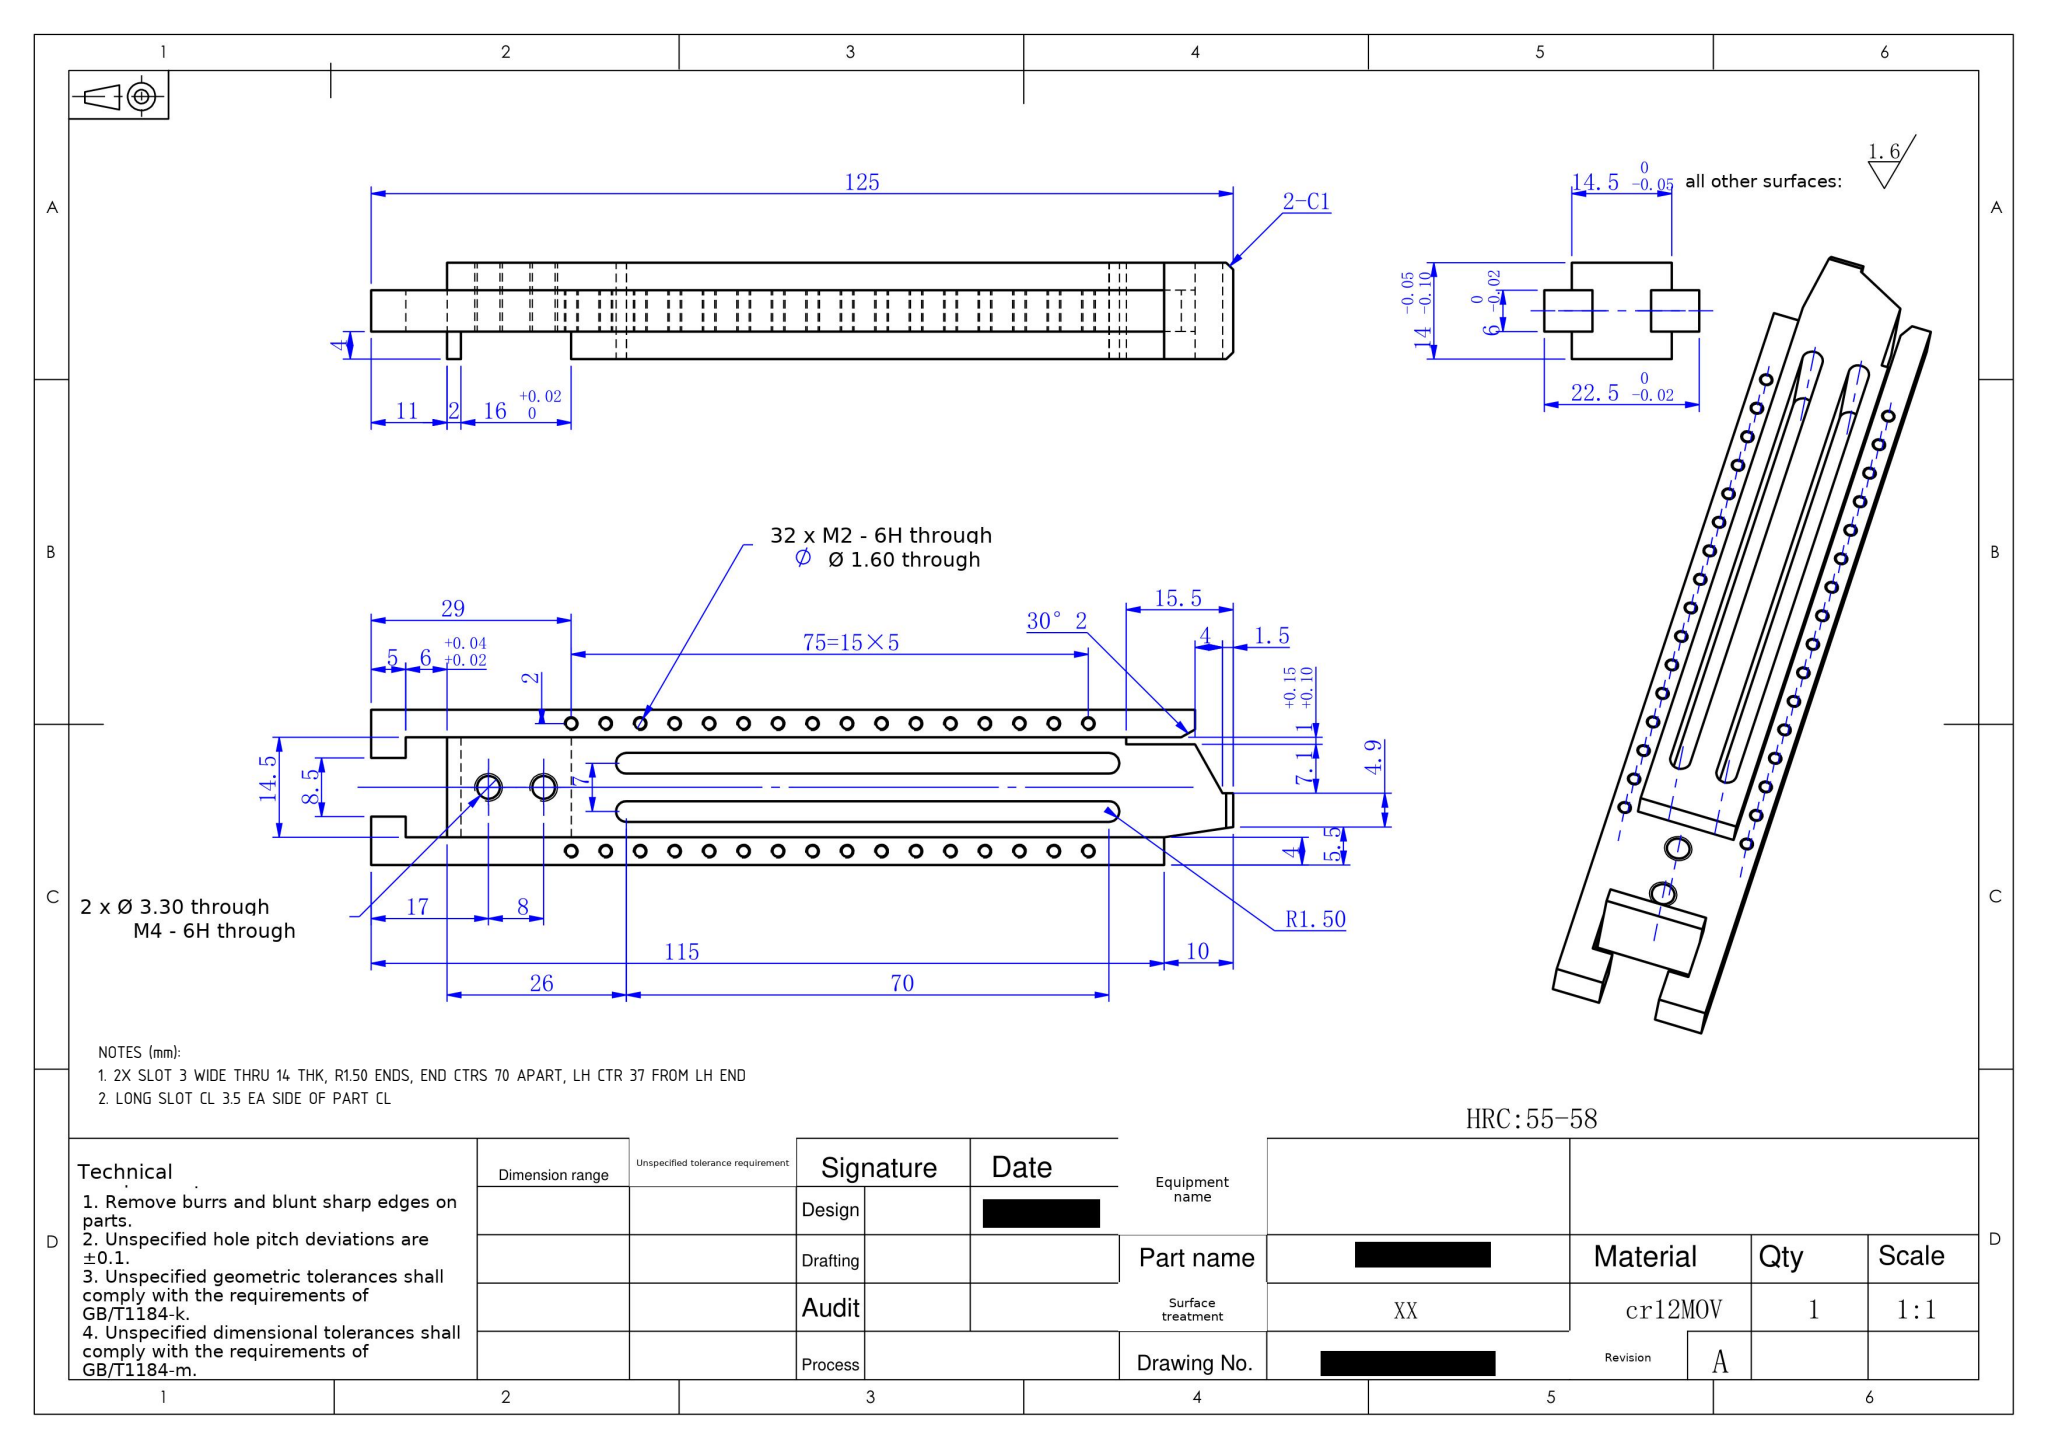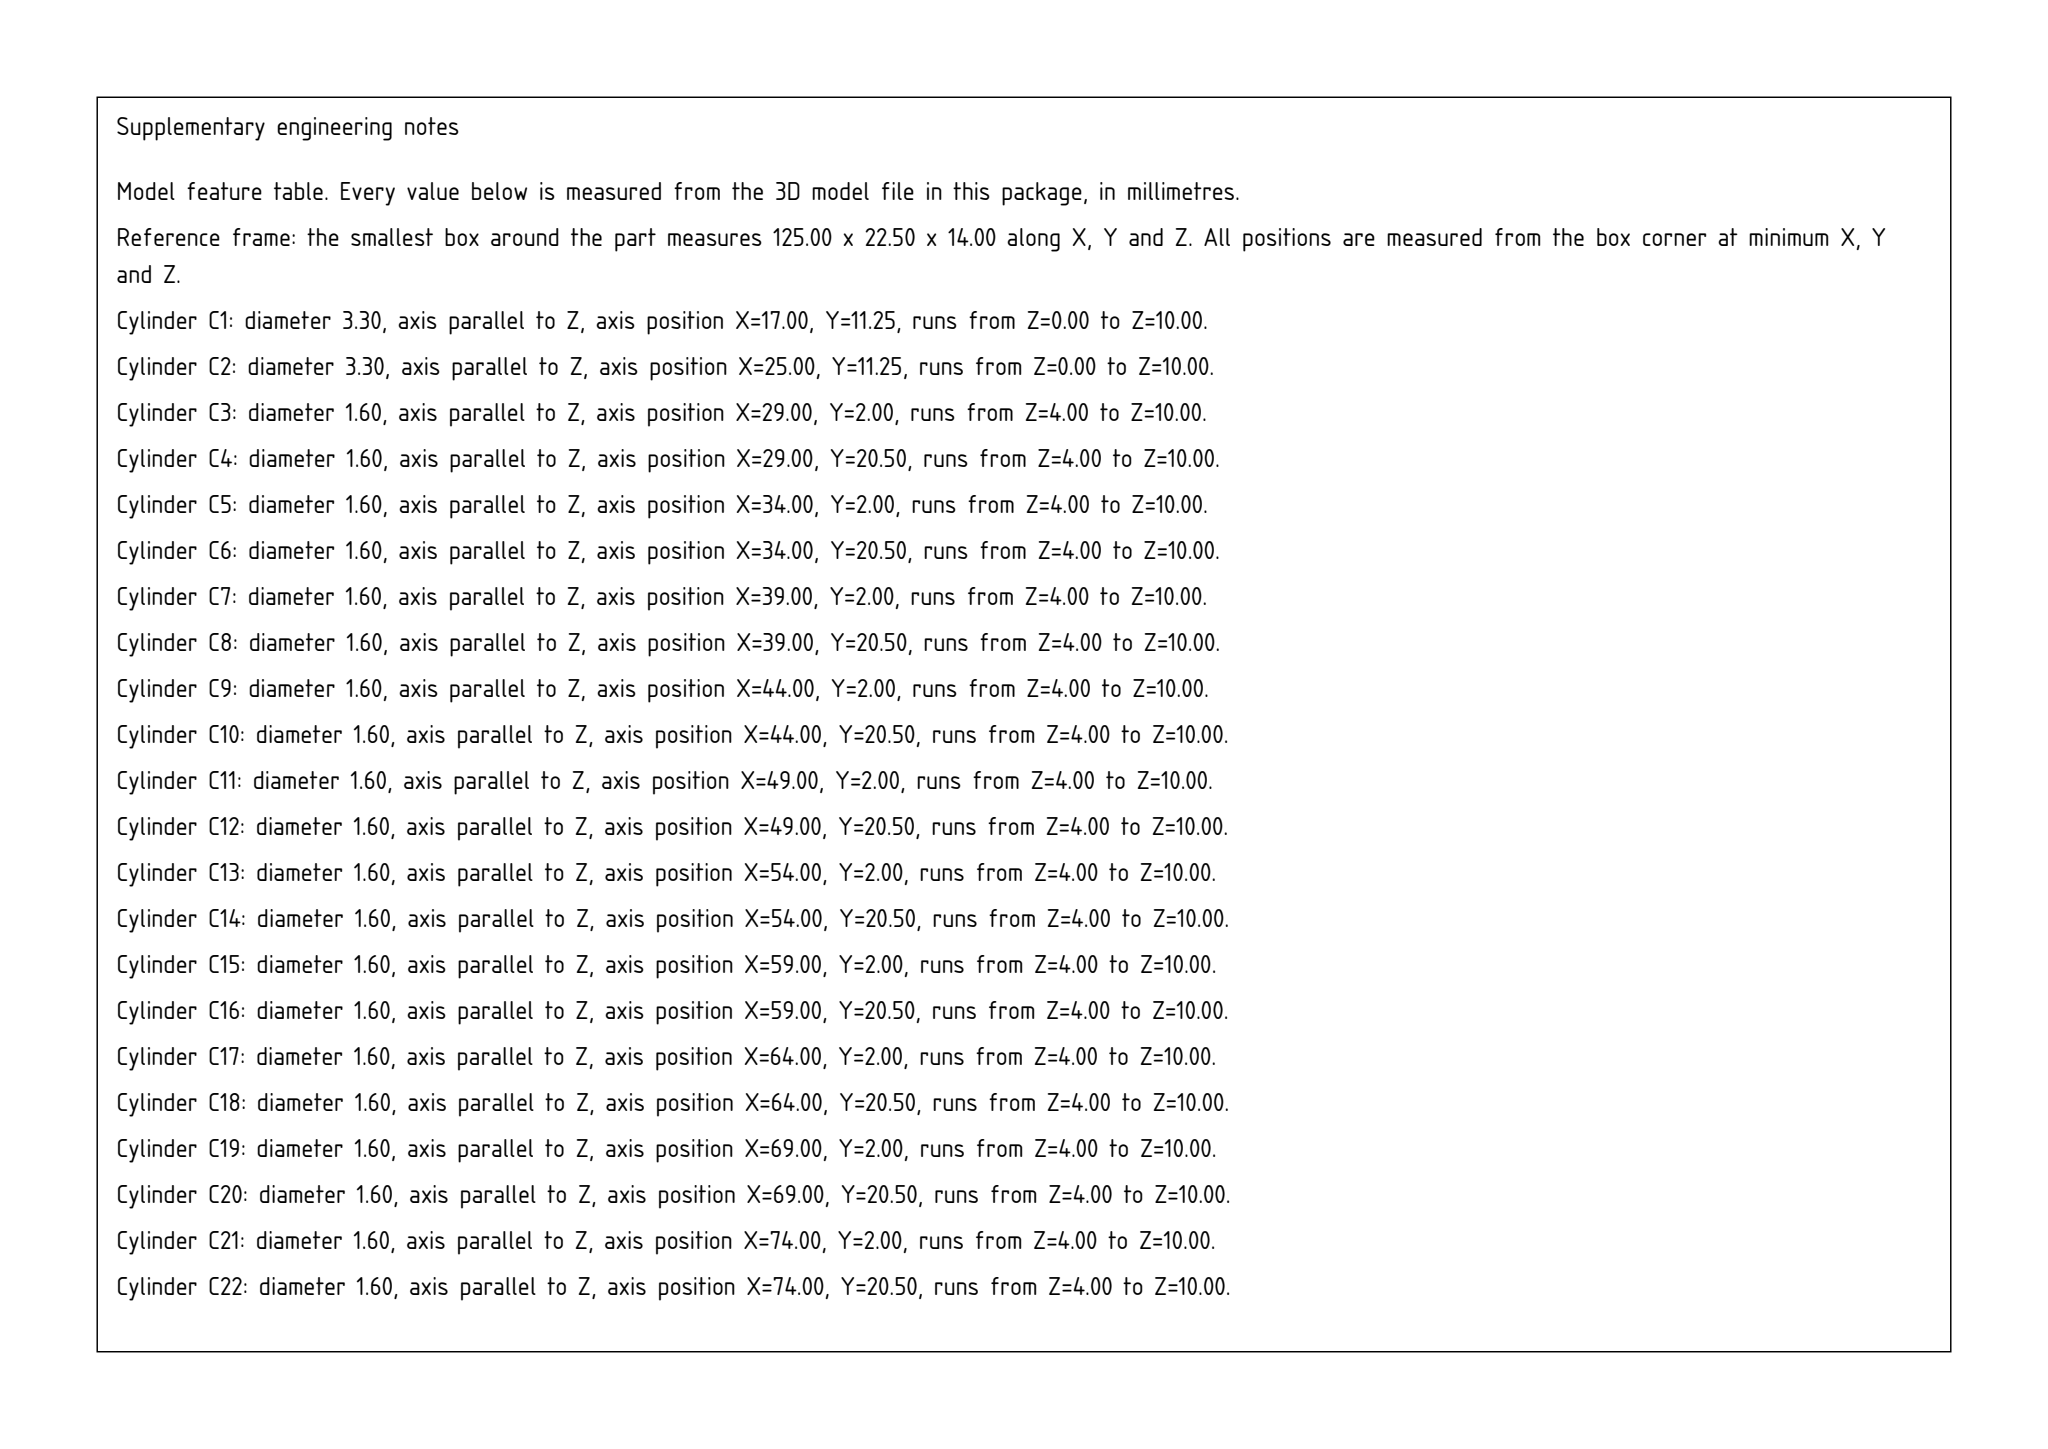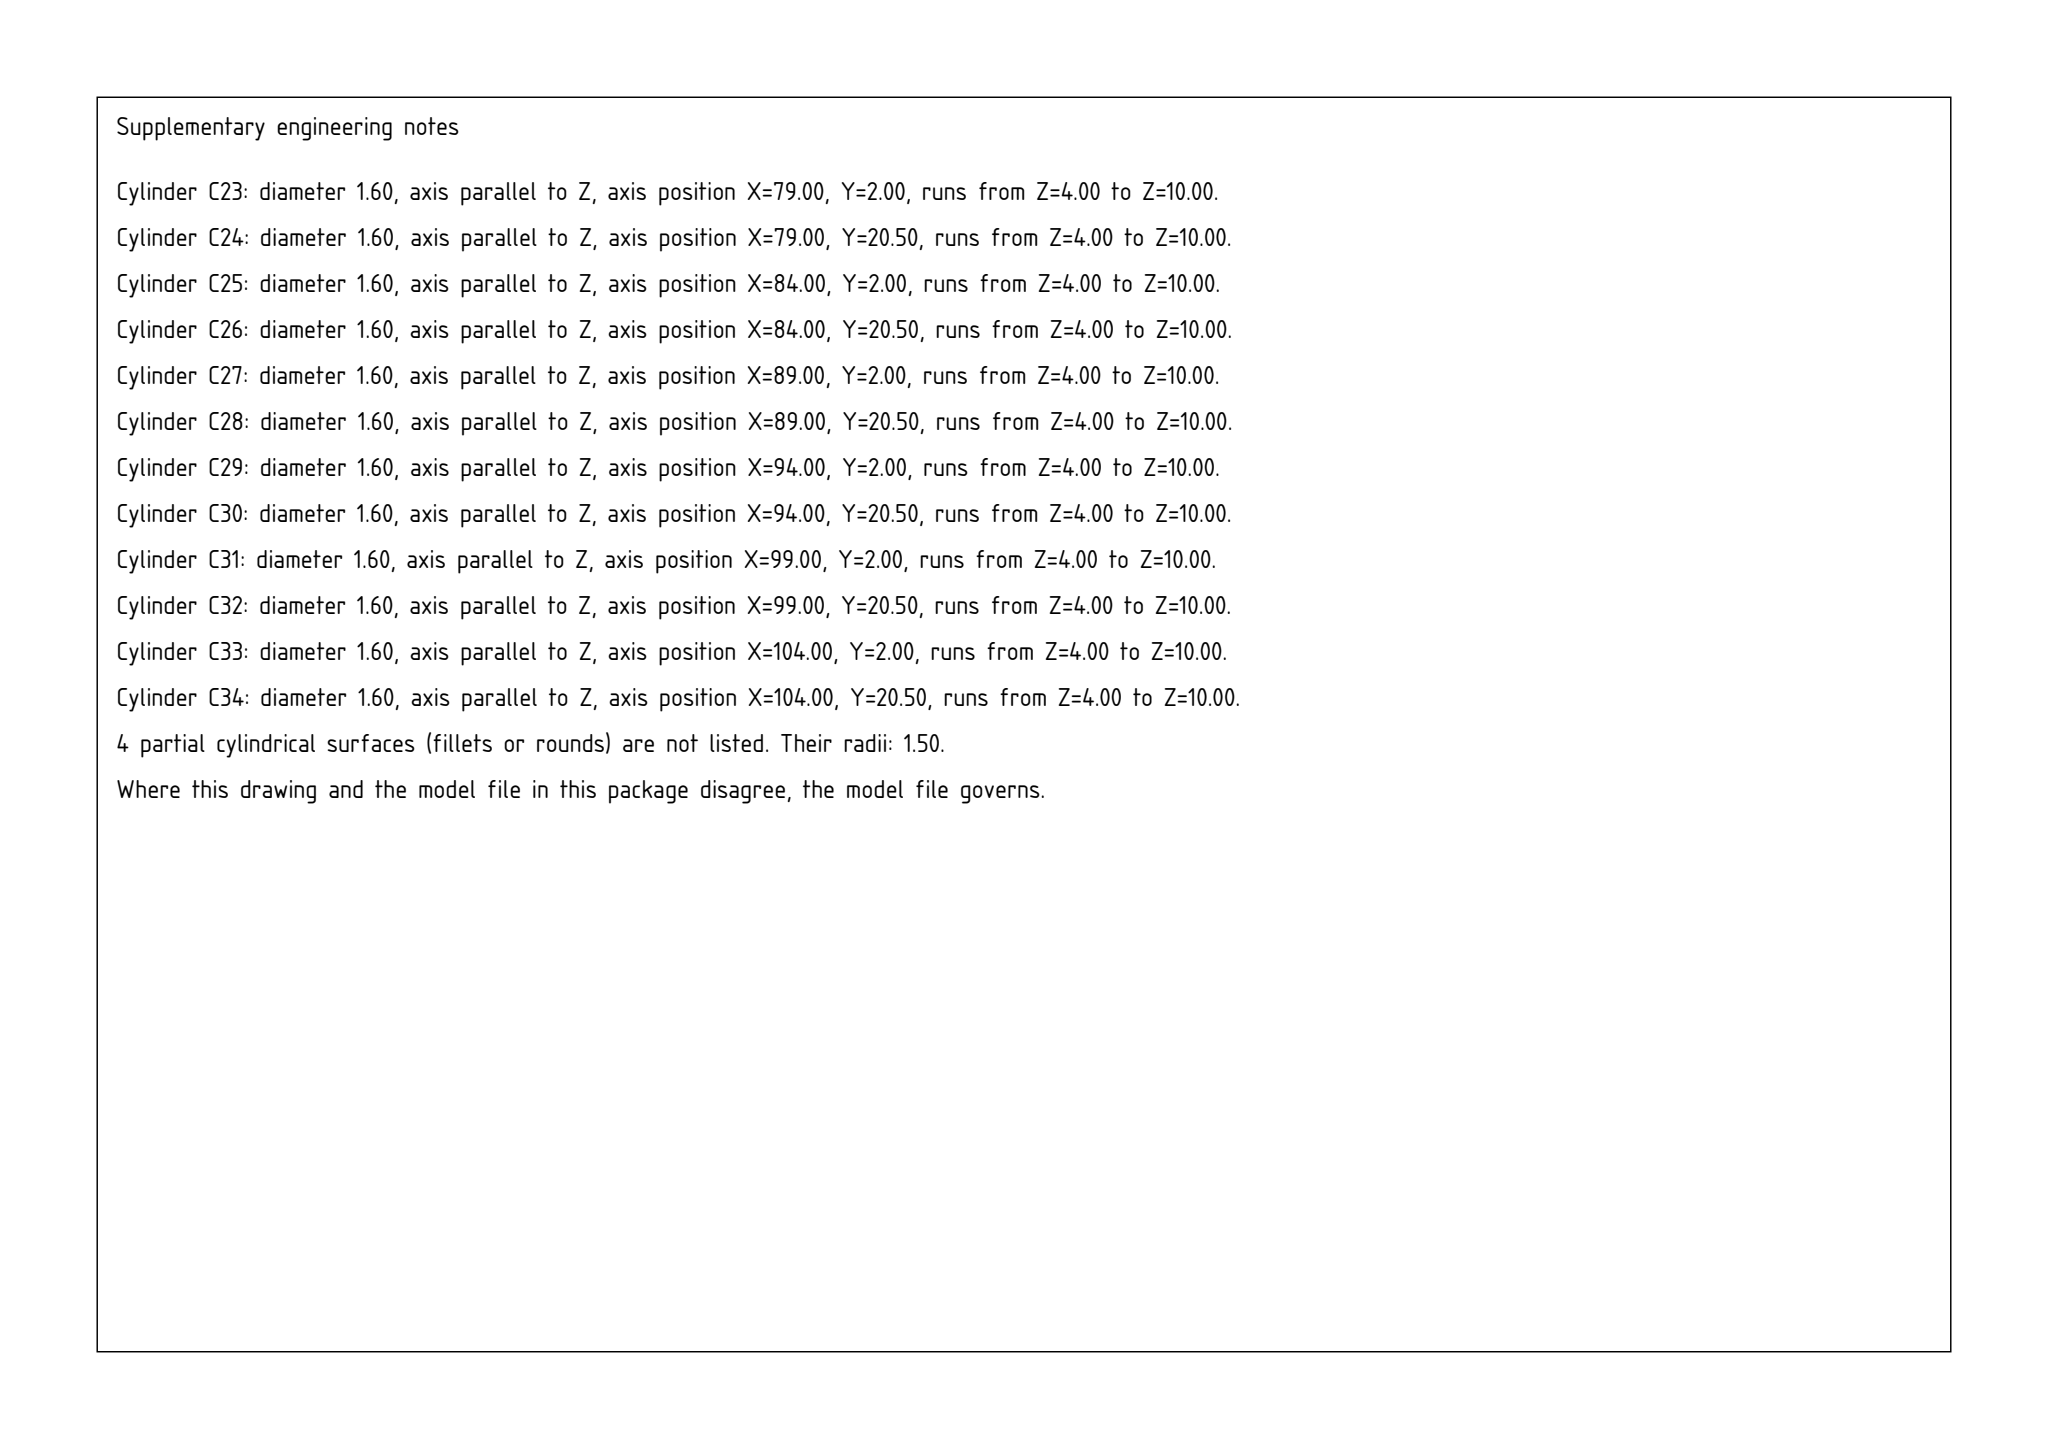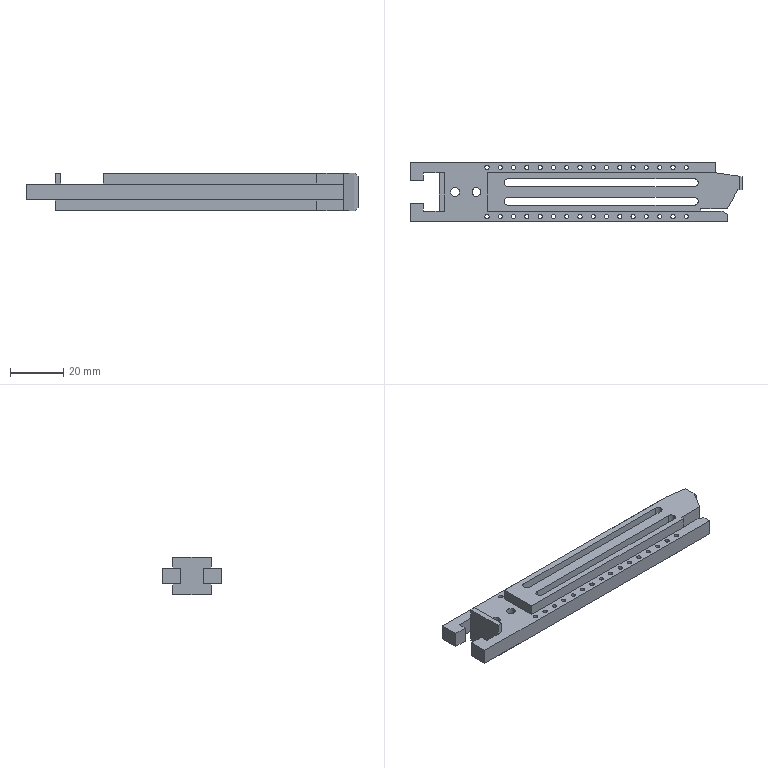Part | SolidWorks | mm | 1 solid | 115 faces | box 125 x 22.5 x 14 mm | volume 20702 mm3 | cylinder 74 | plane 41 | commonest cylinder face diameters 1.6 x64 3 x6 3.3 x4
Drawing notes:
2X SLOT 3 WIDE THRU 14 THK, R1.50 ENDS, END CTRS 70 APART, LH CTR 37 FROM LH END | from the solid: Ø3.0 z-cyls at x=37 & x=107, y=7.75/14.75, length 14 = full thk; z planes 0 & 14
LONG SLOT CL 3.5 EA SIDE OF PART CL | from the solid: slot axes y=7.75 & 14.75; bbox y=22.5 -> CL y=11.25, +/-3.5
build123d program:
from build123d import *

# Parameters (mm, degrees)
SKETCH1_W           = 125
SKETCH1_H           = 14.5
BOSS_EXTRUDE1_DEPTH = 14
CUT_EXTRUDE1_DEPTH  = 71.902
SKETCH3_W           = 119.47
SKETCH3_H           = 6
BOSS_EXTRUDE2_DEPTH = 4
CHAMFER1_SIZE       = 2
CHAMFER1_SIZE2      = 1.155
CHAMFER2_SIZE       = 1
SKETCH4_W           = 115
SKETCH4_H           = 6
BOSS_EXTRUDE3_DEPTH = 4
CUT_EXTRUDE2_DEPTH  = 72.694
SKETCH6_W           = 11
SKETCH6_H           = 8.5
CUT_EXTRUDE3_DEPTH  = 72.694
SKETCH7_W           = 6
SKETCH7_H           = 14.5
CUT_EXTRUDE4_DEPTH  = 72.694
SKETCH9_W           = 5
SKETCH9_H           = 4
CUT_EXTRUDE5_DEPTH  = 73.265
SKETCH10_W          = 16
SKETCH10_H          = 4
CUT_EXTRUDE6_DEPTH  = 73.265
M4_TAPPED_HOLE1_D   = 3.3
CUT_EXTRUDE7_DEPTH  = 72.694
M2_TAPPED_HOLE1_D   = 1.6


with BuildPart() as part:
    # Sketch1 → Boss-Extrude1 (new body)
    with BuildSketch(Plane.XY):
        with Locations((5.939, 4.878)):
            Rectangle(SKETCH1_W, SKETCH1_H)
    extrude(amount=BOSS_EXTRUDE1_DEPTH)

    # Sketch2 → Cut-Extrude1 (cut, through all)
    with BuildSketch(Plane.XY.offset(14)):
        Polygon((52.939, -2.372), (52.939, -1.372), (62.91, -1.372), (66.91, 5.728), (68.439, 5.728), (68.439, -2.372), align=None)
    extrude(amount=-CUT_EXTRUDE1_DEPTH, mode=Mode.SUBTRACT)

    # Sketch3 → Boss-Extrude2 (add)
    with BuildSketch(Plane(origin=(0, -2.372, 0), x_dir=(-1, 0, 0), z_dir=(0, -1, 0))):
        with Locations((-3.175, -7)):
            Rectangle(SKETCH3_W, SKETCH3_H)
    extrude(amount=BOSS_EXTRUDE2_DEPTH)

    # Chamfer1
    chamfer1_edges = [part.edges().sort_by_distance(p)[0] for p in [
        (62.91, -2.372, 7),
    ]]
    chamfer1_side = [part.faces().sort_by_distance(p)[0] for p in [
        (57.925, -2.372, 7),
    ]]
    chamfer(chamfer1_edges, length=CHAMFER1_SIZE, length2=CHAMFER1_SIZE2, reference=chamfer1_side[0])

    # Chamfer2
    chamfer2_edges = [part.edges().sort_by_distance(p)[0] for p in [
        (68.439, 8.928, 0),
        (68.439, 8.928, 14),
    ]]
    chamfer(chamfer2_edges, length=CHAMFER2_SIZE)

    # Sketch4 → Boss-Extrude3 (add)
    with BuildSketch(Plane(origin=(0, 12.128, 0), x_dir=(1, 0, 0), z_dir=(0, 1, 0))):
        with Locations((0.9393, -7)):
            Rectangle(SKETCH4_W, SKETCH4_H)
    extrude(amount=BOSS_EXTRUDE3_DEPTH)

    # Sketch5 → Cut-Extrude2 (cut, through all)
    with BuildSketch(Plane.XY.offset(14)):
        Polygon((58.439, 12.128), (68.439, 10.628), (68.439, 12.128), align=None)
    extrude(amount=-CUT_EXTRUDE2_DEPTH, mode=Mode.SUBTRACT)

    # Sketch6 → Cut-Extrude3 (cut, through all)
    with BuildSketch(Plane.XY.offset(14)):
        with Locations((-51.061, 4.878)):
            Rectangle(SKETCH6_W, SKETCH6_H)
    extrude(amount=-CUT_EXTRUDE3_DEPTH, mode=Mode.SUBTRACT)

    # Sketch7 → Cut-Extrude4 (cut, through all)
    with BuildSketch(Plane.XY.offset(14)):
        with Locations((-48.561, 4.878)):
            Rectangle(SKETCH7_W, SKETCH7_H)
    extrude(amount=-CUT_EXTRUDE4_DEPTH, mode=Mode.SUBTRACT)

    # Sketch9 → Cut-Extrude5 (cut, through all)
    with BuildSketch(Plane(origin=(0, 12.128, 0), x_dir=(1, 0, 0), z_dir=(0, 1, 0))):
        with Locations((-54.061, -2)):
            Rectangle(SKETCH9_W, SKETCH9_H)
        with Locations((-54.061, -12)):
            Rectangle(SKETCH9_W, SKETCH9_H)
    extrude(amount=-CUT_EXTRUDE5_DEPTH, mode=Mode.SUBTRACT)

    # Sketch10 → Cut-Extrude6 (cut, through all)
    with BuildSketch(Plane(origin=(0, 12.128, 0), x_dir=(1, 0, 0), z_dir=(0, 1, 0))):
        with Locations((-35.561, -12)):
            Rectangle(SKETCH10_W, SKETCH10_H)
    extrude(amount=-CUT_EXTRUDE6_DEPTH, mode=Mode.SUBTRACT)

    # M4 Tapped Hole1 (through all)
    with Locations(Plane.XY.offset(10)):
        with Locations((-31.561, 4.878), (-39.561, 4.878)):
            Hole(M4_TAPPED_HOLE1_D / 2)

    # Sketch13 → Cut-Extrude7 (cut, through all)
    with BuildSketch(Plane.XY.offset(14)):
        with BuildLine():
            Line((-19.561, 9.878), (50.439, 9.878))
            ThreePointArc((50.439, 9.878), (51.939, 8.378), (50.439, 6.878))
            Line((50.439, 6.878), (-19.561, 6.878))
            ThreePointArc((-19.561, 6.878), (-21.061, 8.378), (-19.561, 9.878))
        make_face()
        with BuildLine():
            Line((-19.561, 2.878), (50.439, 2.878))
            ThreePointArc((50.439, 2.878), (51.939, 1.378), (50.439, -0.1219))
            Line((50.439, -0.1219), (-19.561, -0.1219))
            ThreePointArc((-19.561, -0.1219), (-21.061, 1.378), (-19.561, 2.878))
        make_face()
    extrude(amount=-CUT_EXTRUDE7_DEPTH, mode=Mode.SUBTRACT)

    # M2 Tapped Hole1 (through all)
    with Locations(Plane.XY.offset(10)):
        with Locations((-22.561, 14.128), (-17.561, 14.128), (-12.561, 14.128), (-7.561, 14.128), (-2.561, 14.128), (2.439, 14.128), (7.439, 14.128), (12.439, 14.128), (17.439, 14.128), (22.439, 14.128), (27.439, 14.128), (32.439, 14.128), (37.439, 14.128), (42.439, 14.128), (47.439, 14.128), (-27.561, 14.128), (-27.561, -4.372), (47.439, -4.372), (42.439, -4.372), (37.439, -4.372), (32.439, -4.372), (27.439, -4.372), (22.439, -4.372), (17.439, -4.372), (12.439, -4.372), (7.439, -4.372), (2.439, -4.372), (-2.561, -4.372), (-7.561, -4.372), (-12.561, -4.372), (-17.561, -4.372), (-22.561, -4.372)):
            Hole(M2_TAPPED_HOLE1_D / 2)


solid = part.part